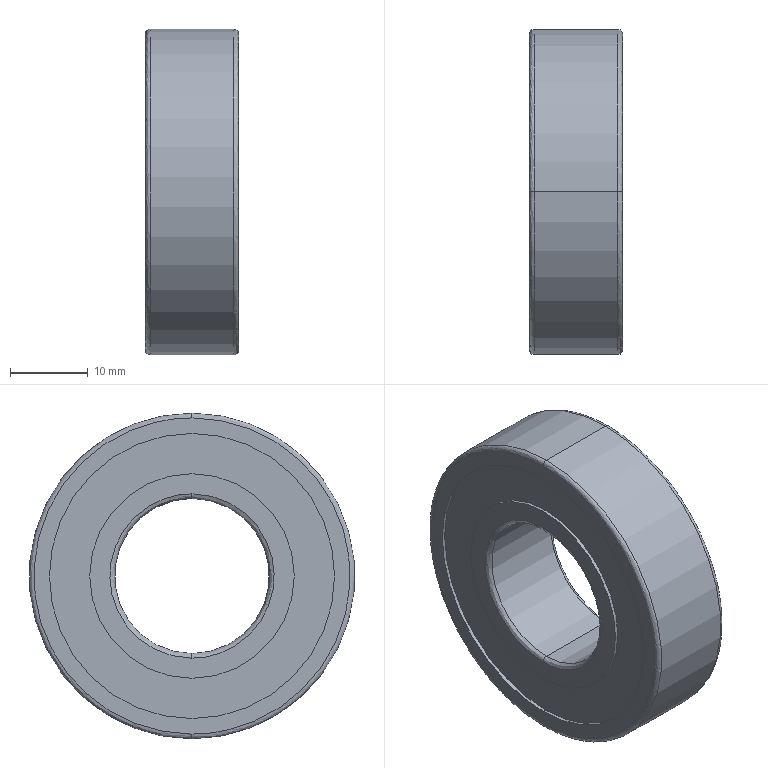Component | SolidWorks | BAY6004ZZBearing-1 | 1 solid | 26 faces | volume 12380 mm3 | cylinder 12 | spline 8 | plane 6 | commonest cylinder face diameters 36.8 x4 26.4 x4 42 x2 20 x2